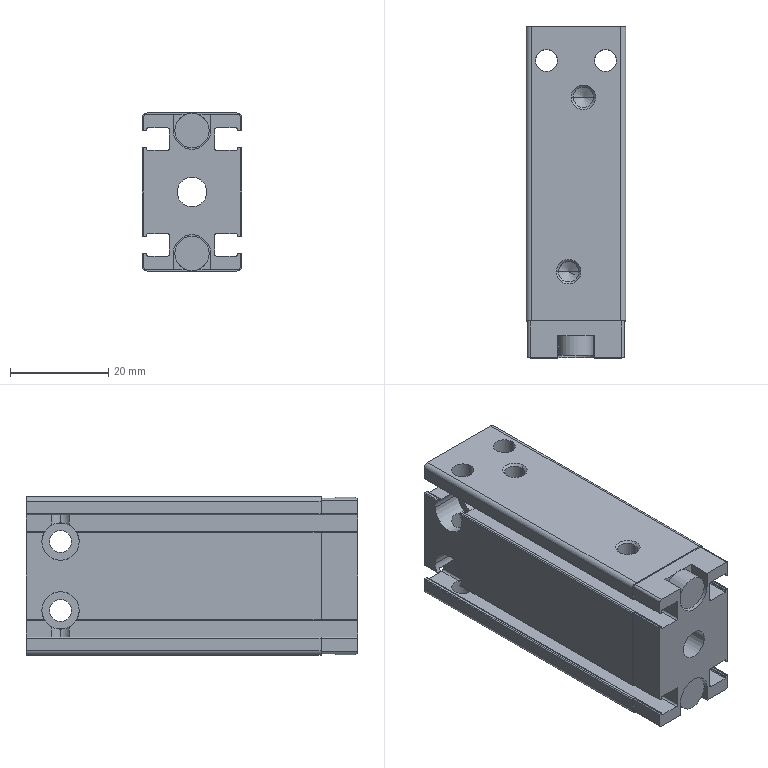Component | SolidWorks | MDJ16x20-10S_00_+-1_MDJ16x20-10S_00_+_1-1 | 1 solid | 210 faces | volume 28350 mm3 | cylinder 112 | plane 82 | cone 16 | commonest cylinder face diameters 0.4 x44 4.5 x16 0.8 x16 7.6 x10 6 x4 3.242 x4 4.134 x4 7 x4